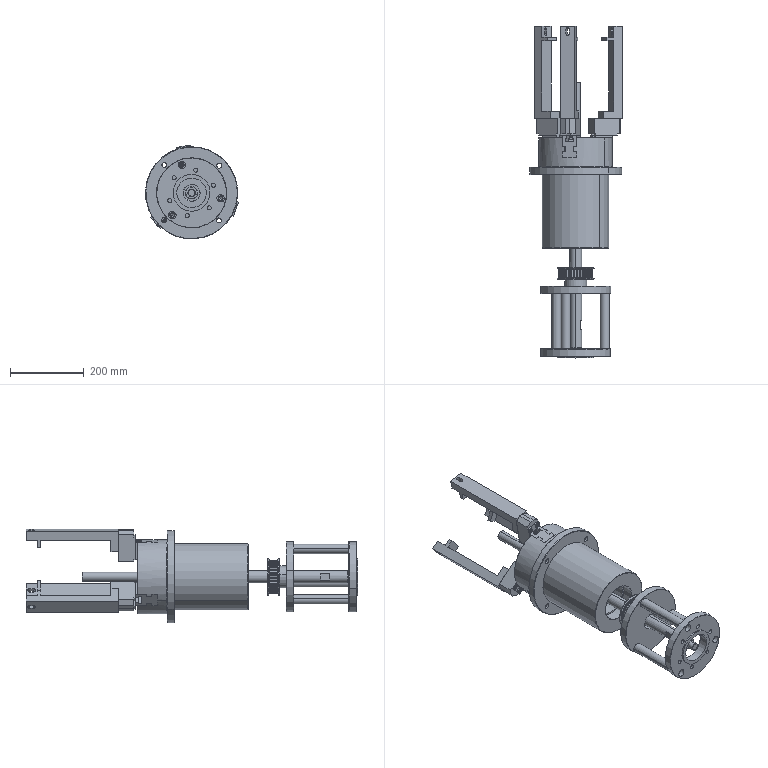Assembly | SolidWorks | mm | 20 component files | 22 solids | 2114 faces | box 251.89 x 898.82 x 254.42 mm | volume 8661204 mm3 | plane 1626 | cylinder 399 | cone 89 | commonest cylinder face diameters 1.81 x90 4.8 x53 20 x50 90.302 x36 13.5 x32 13 x18 18 x14 11 x12
Bill of materials:
009A-20130717 | 1 |  | Flat circular flange disc with a central through bore, a short cylindrical boss on one face around the bore, and three small through holes evenly spaced near the rim.
010A-20130717 | 1 |  | Annular flange plate with a large central bore, a thin raised spigot ring on one face, and nine through holes on a bolt circle: three larger and six smaller.
011A-20130717 | 3 |  | Plain cylindrical tube or sleeve with a small concentric axial bore and flat square-cut ends.
008A-20130717 | 1 |  | Flanged cylindrical sleeve: a thick-walled tubular body with a through bore and a thin circular flange at one end with four small through holes.
012A-20130717 | 1 |  | Slender stepped round shaft: a long main diameter that steps down near one end to a short smaller-diameter pin, with a small flat or keyseat-like patch near the stepped end.
026A-20130717 | 1 |  | Cylindrical rod fixed at right angles to a thin plate with a roughly three-lobed outline. The plate has three hook-like notches in its edge, three small through holes, and a circular feature at its centre where the rod meets it.
HTS8-36-20A | 1 |  | Toothed wheel with many evenly spaced axial teeth around a cylindrical body, a flange with a chamfered outer edge on each side, and a central bore with one keyway.
K51-1 | 1 |  | Thick annular ring with a large central bore. It has six axial through holes arranged in three pairs, stepped T-shaped slots in the outer surface, rectangular notches in the bore, and a recessed step on one face.
K51-2 | 3 |  | Irregular prismatic block: a mostly rectangular body with a T-shaped tab (narrow neck, wider head) projecting from one side, several stepped rectangular notches, and at least one sloped face.
K51-3 | 1 |  | Solid circular disc with three T-shaped slots cut inward from the outer edge through the full thickness, spaced roughly evenly around the circumference.
K51-4 | 3 |  | Rectangular block with one end clipped by two chamfers, two round through holes, and finely serrated strips on one face on either side of the holes, plus a stepped tongue along the base.
K51-5 | 3 |  | Long rectangular bar with a downward leg at one end and a shorter downward tab near the other end. It has a round hole in the end face of the leg end and an elongated slot through the bar near the opposite end.
Mates:
1. coincident | HTS8-36-20A-1 face at (-240, 617.678, 90) dir (0, -1, 0) | 002AS-20130718-1/009A-20130717-1 face at (-240, 617.678, 90) dir (0, 1, 0)
2. concentric | assembly face at (-240, 918, 90) dir (0, 1, 0) r 75 | 008A-20130717-1 face at (-240, 873, 90) dir (0, 1, 0) r 75
3. coincident | assembly face at (-309.466, 873, 110.755) dir (0, -1, 0) | 008A-20130717-1 face at (-240, 873, 90) dir (0, 1, 0)
4. coincident | K51-2/K51-1-1 face at (-240, 1000, 90) dir (0, 1, 0) | 026A-20130717-1 face at (-240, 1000, 90) dir (0, 1, 0)
5. concentric | K51-2/K51-1-1 face at (-240, 1000, 90) dir (0, -1, 0) r 100 | 026A-20130717-1 face at (-240, 1150, 90) dir (0, -1, 0) r 12.5
6. parallel | 026A-20130717-1 face at (-187.238, 996, 48.129) dir (0.3464, 0, 0.9381) | K51-2/K51-2-3 face at (-185.81, 976.5, 91.308) dir (0.3464, 0, 0.9381)
7. concentric | 009A-20130717-1 face at (0, 20, 0) dir (0, -1, 0) r 95 | 010A-20130717-1 face at (0, -170, 0) dir (0, 1, 0) r 95
8. coincident | 009A-20130717-1 face at (0, 0, 0) dir (0, -1, 0) | 011A-20130717-2 face at (0, 0, -80) dir (0, 1, 0)
9. coincident | 009A-20130717-1 face at (0, 0, 0) dir (0, -1, 0) | 011A-20130717-3 edge at (69.282, 0, 40) dir (0, 1, 0) r 12
10. coincident | 009A-20130717-1 face at (0, 0, 0) dir (0, -1, 0) | 011A-20130717-4 face at (-69.282, 0, 40) dir (0, 1, 0)
11. concentric | 009A-20130717-1 face at (0, 20, -80) dir (0, 1, 0) r 10 | 011A-20130717-2 face at (0, 0, -80) dir (0, 1, 0) r 5.25
12. concentric | 009A-20130717-1 face at (69.282, 20, 40) dir (0, 1, 0) r 10 | 011A-20130717-3 face at (69.282, 0, 40) dir (0, 1, 0) r 5.25
13. concentric | 009A-20130717-1 face at (-69.282, 20, 40) dir (0, 1, 0) r 10 | 011A-20130717-4 face at (-69.282, 0, 40) dir (0, -1, 0) r 12.5
14. concentric | 010A-20130717-1 face at (69.282, -170, 40) dir (0, -1, 0) r 6.75 | 011A-20130717-3 face at (69.282, 0, 40) dir (0, -1, 0) r 12.5
15. coincident | K51-1-1 face at (-20, 26.5, -30) dir (0, 1, 0) | K51-2-1 face at (-20, 26.5, -50.382) dir (0, -1, 0)
16. coincident | K51-1-1 face at (12.25, 41.5, -30) dir (-1, 0, 0) | K51-2-1 face at (12.25, 41.5, -50.382) dir (1, 0, 0)
17. coincident | K51-1-1 face at (-15.981, 26.5, 32.321) dir (0, 1, 0) | K51-2-2 face at (-33.632, 26.5, 42.511) dir (0, -1, 0)
18. coincident | K51-1-1 face at (-19.856, 41.5, 25.609) dir (-0.5, 0, -0.866) | K51-2-2 face at (-37.507, 41.5, 35.8) dir (0.5, 0, 0.866)
19. coincident | K51-1-1 face at (35.981, 26.5, -2.321) dir (0, 1, 0) | K51-2-3 face at (53.632, 26.5, 7.87) dir (0, -1, 0)
20. coincident | K51-1-1 face at (19.856, 41.5, 25.609) dir (0.5, 0, -0.866) | K51-2-3 face at (37.507, 41.5, 35.8) dir (-0.5, 0, 0.866)
21. concentric | K51-1-1 face at (0, 0, 0) dir (0, 1, 0) r 50 | K51-3-1 face at (0, 68.664, 0) dir (0, -1, 0) r 45
22. coincident | K51-2-3 face at (40.69, -43.106, 14.832) dir (-0.8529, -0.1736, -0.4924) | K51-3-1 face at (34.846, -4.834, 11.458) dir (0.8529, 0.1736, 0.4924)
23. coincident | K51-2-1 face at (-7.5, -43.106, -42.655) dir (0, -0.1736, 0.9848) | K51-3-1 face at (-7.5, -4.834, -35.907) dir (0, 0.1736, -0.9848)
24. coincident | K51-2-2 face at (-33.19, -43.106, 27.823) dir (0.8529, -0.1736, -0.4924) | K51-3-1 face at (-27.346, -4.834, 24.448) dir (-0.8529, 0.1736, 0.4924)
25. coincident | K51-2-3 face at (33.632, 56.5, 42.511) dir (-0.5, 0, 0.866) | K51-4-1 face at (100.749, 86, 81.261) dir (-0.5, 0, 0.866)
26. coincident | K51-2-3 face at (54.065, 86.5, 8.12) dir (0.6124, 0.7071, 0.3536) | K51-4-1 face at (75.065, 86.5, -28.253) dir (-0.6124, -0.7071, -0.3536)
27. coincident | K51-2-3 face at (54.498, 86, 8.37) dir (-0.6124, 0.7071, -0.3536) | K51-4-1 face at (75.498, 86, -28.003) dir (0.6124, -0.7071, 0.3536)
28. coincident | K51-2-2 face at (-33.632, 56.5, 42.511) dir (0.5, 0, 0.866) | K51-4-3 face at (-100.749, 132, 81.261) dir (0.5, 0, 0.866)
29. coincident | K51-2-2 face at (-34.065, 86.5, 42.761) dir (-0.6124, 0.7071, 0.3536) | K51-4-3 face at (-13.065, 86.5, 79.134) dir (0.6124, -0.7071, -0.3536)
30. coincident | K51-2-2 face at (-34.498, 86, 43.011) dir (0.6124, 0.7071, -0.3536) | K51-4-3 face at (-13.498, 86, 79.384) dir (-0.6124, -0.7071, 0.3536)
31. coincident | K51-2-1 face at (-20, 86.5, -50.882) dir (0, 0.7071, -0.7071) | K51-4-2 face at (-62, 86.5, -50.882) dir (0, -0.7071, 0.7071)
32. coincident | K51-2-1 face at (-20, 86, -51.382) dir (0, 0.7071, 0.7071) | K51-4-2 face at (-62, 86, -51.382) dir (0, -0.7071, -0.7071)
33. coincident | K51-2-1 face at (-20, 56.5, -50.382) dir (-1, 0, 0) | K51-4-2 face at (-20, 132, -127.882) dir (-1, 0, 0)
34. coincident | K51-4-3 face at (-110.749, 90, 63.941) dir (-0.866, 0, 0.5) | K51-5-1 face at (-100.749, 132, 81.261) dir (-0.866, 0, 0.5)
35. coincident | K51-4-3 face at (-120.749, 86, 46.62) dir (-0.5, 0, -0.866) | K51-5-1 face at (-120.749, 132, 46.62) dir (-0.5, 0, -0.866)
36. coincident | K51-4-3 face at (-120.749, 132, 46.62) dir (0, 1, 0) | K51-5-1 face at (-53.117, 132, 53.761) dir (0, -1, 0)
37. coincident | K51-4-2 face at (20, 132, -127.882) dir (0, 1, 0) | K51-5-2 face at (-20, 132, -72.882) dir (0, -1, 0)
38. concentric | K51-4-2 face at (0, 132, -84.882) dir (0, 1, 0) r 10 | K51-5-2 face at (0, 122, -84.882) dir (0, 1, 0) r 6.5
39. coincident | K51-4-2 face at (-20, 132, -127.882) dir (-1, 0, 0) | K51-5-2 face at (-20, 132, -127.882) dir (-1, 0, 0)
40. coincident | K51-4-1 face at (100.749, 132, 81.261) dir (0, 1, 0) | K51-5-3 face at (73.117, 132, 19.12) dir (0, -1, 0)
41. concentric | K51-4-1 face at (73.51, 132, 42.441) dir (0, 1, 0) r 10 | K51-5-3 face at (73.51, 122, 42.441) dir (0, 1, 0) r 6.5
42. coincident | K51-4-1 face at (110.749, 90, 63.941) dir (0.866, 0, 0.5) | K51-5-3 face at (120.749, 132, 46.62) dir (0.866, 0, 0.5)